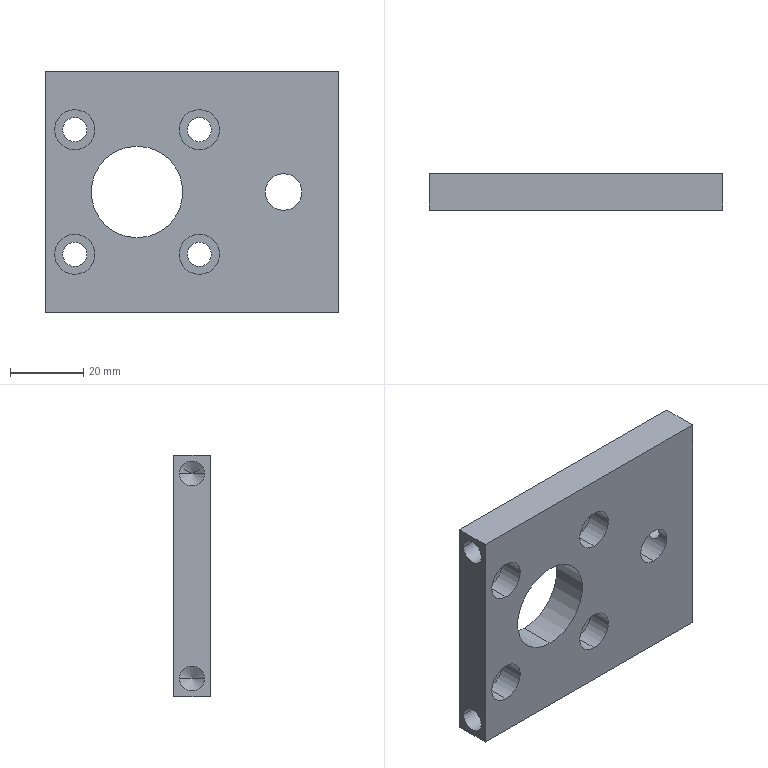Component | SolidWorks | SHYTJ-01-07-06CylinderMountingPlate-1 | 1 solid | 40 faces | box 80 x 10 x 66 mm | volume 42459 mm3 | cylinder 26 | plane 10 | cone 4 | commonest cylinder face diameters 11 x8 6.6 x8 6.8 x4 4.2 x2 10 x2 25 x2
build123d program:
from build123d import *

# Parameters (mm, degrees)
SKETCH1_W                                         = 66
SKETCH1_H                                         = 80
SKETCH1_R                                         = 12.5
BOSS_EXTRUDE1_DEPTH                               = 10
M8_TAPPED_HOLE1_D                                 = 6.8
M8_TAPPED_HOLE1_DEPTH                             = 19.75
M8_TAPPED_HOLE1_TIP                               = 2.043
HOLE_SIZE_ACCORDING_TO_TYPE_OF_SOCKET_D           = 6.6
HOLE_SIZE_ACCORDING_TO_TYPE_OF_SOCKET_DEPTH       = 19.75
HOLE_SIZE_ACCORDING_TO_TYPE_OF_SOCKET_CBORE_D     = 11
HOLE_SIZE_ACCORDING_TO_TYPE_OF_SOCKET_CBORE_DEPTH = 6.8
HOLE_SIZE_ACCORDING_TO_TYPE_OF_SOCKET_TIP         = 1.983
SKETCH7_R                                         = 5
CUT_EXTRUDE1_DEPTH                                = 10
M5_TAPPED_HOLE1_D                                 = 4.2
M5_TAPPED_HOLE1_DEPTH                             = 12.4
M5_TAPPED_HOLE1_TIP                               = 1.262


with BuildPart() as part:
    # Sketch1 → Boss-Extrude1 (new body)
    with BuildSketch(Plane.XY):
        with Locations((0, 15)):
            Rectangle(SKETCH1_W, SKETCH1_H)
        Circle(SKETCH1_R, mode=Mode.SUBTRACT)
    extrude(amount=BOSS_EXTRUDE1_DEPTH)

    # M8 Tapped Hole1
    with Locations(Plane(origin=(0, -25, 0), x_dir=(-1, 0, 0), z_dir=(0, -1, 0))):
        with Locations((28, -5), (-28, -5)):
            Hole(M8_TAPPED_HOLE1_D / 2, depth=M8_TAPPED_HOLE1_DEPTH)
            with Locations((0, 0, -(M8_TAPPED_HOLE1_DEPTH + M8_TAPPED_HOLE1_TIP / 2))):  # 118° drill point
                Cone(0, M8_TAPPED_HOLE1_D / 2, M8_TAPPED_HOLE1_TIP, mode=Mode.SUBTRACT)

    # Hole Size _according to_ type of socket
    with Locations(Plane.XY.offset(10)):
        with Locations((-17, 17), (17, 17), (17, -17), (-17, -17)):
            CounterBoreHole(HOLE_SIZE_ACCORDING_TO_TYPE_OF_SOCKET_D / 2, HOLE_SIZE_ACCORDING_TO_TYPE_OF_SOCKET_CBORE_D / 2, HOLE_SIZE_ACCORDING_TO_TYPE_OF_SOCKET_CBORE_DEPTH, depth=HOLE_SIZE_ACCORDING_TO_TYPE_OF_SOCKET_DEPTH)
            with Locations((0, 0, -(HOLE_SIZE_ACCORDING_TO_TYPE_OF_SOCKET_DEPTH + HOLE_SIZE_ACCORDING_TO_TYPE_OF_SOCKET_TIP / 2))):  # 118° drill point
                Cone(0, HOLE_SIZE_ACCORDING_TO_TYPE_OF_SOCKET_D / 2, HOLE_SIZE_ACCORDING_TO_TYPE_OF_SOCKET_TIP, mode=Mode.SUBTRACT)

    # Sketch7 → Cut-Extrude1 (cut)
    with BuildSketch(Plane(origin=(0, 0, 0), x_dir=(-1, 0, 0), z_dir=(0, 0, -1))):
        with Locations((0, 40)):
            Circle(SKETCH7_R)
    extrude(amount=-CUT_EXTRUDE1_DEPTH, mode=Mode.SUBTRACT)

    # M5 Tapped Hole1
    with Locations(Plane(origin=(0, 55, 0), x_dir=(1, 0, 0), z_dir=(0, 1, 0))):
        with Locations((0, -5)):
            Hole(M5_TAPPED_HOLE1_D / 2, depth=M5_TAPPED_HOLE1_DEPTH)
            with Locations((0, 0, -(M5_TAPPED_HOLE1_DEPTH + M5_TAPPED_HOLE1_TIP / 2))):  # 118° drill point
                Cone(0, M5_TAPPED_HOLE1_D / 2, M5_TAPPED_HOLE1_TIP, mode=Mode.SUBTRACT)


solid = part.part

# Placed as in the assembly
solid = solid.moved(Location((174.884, -71.361, 270), (90, 0, -90)))